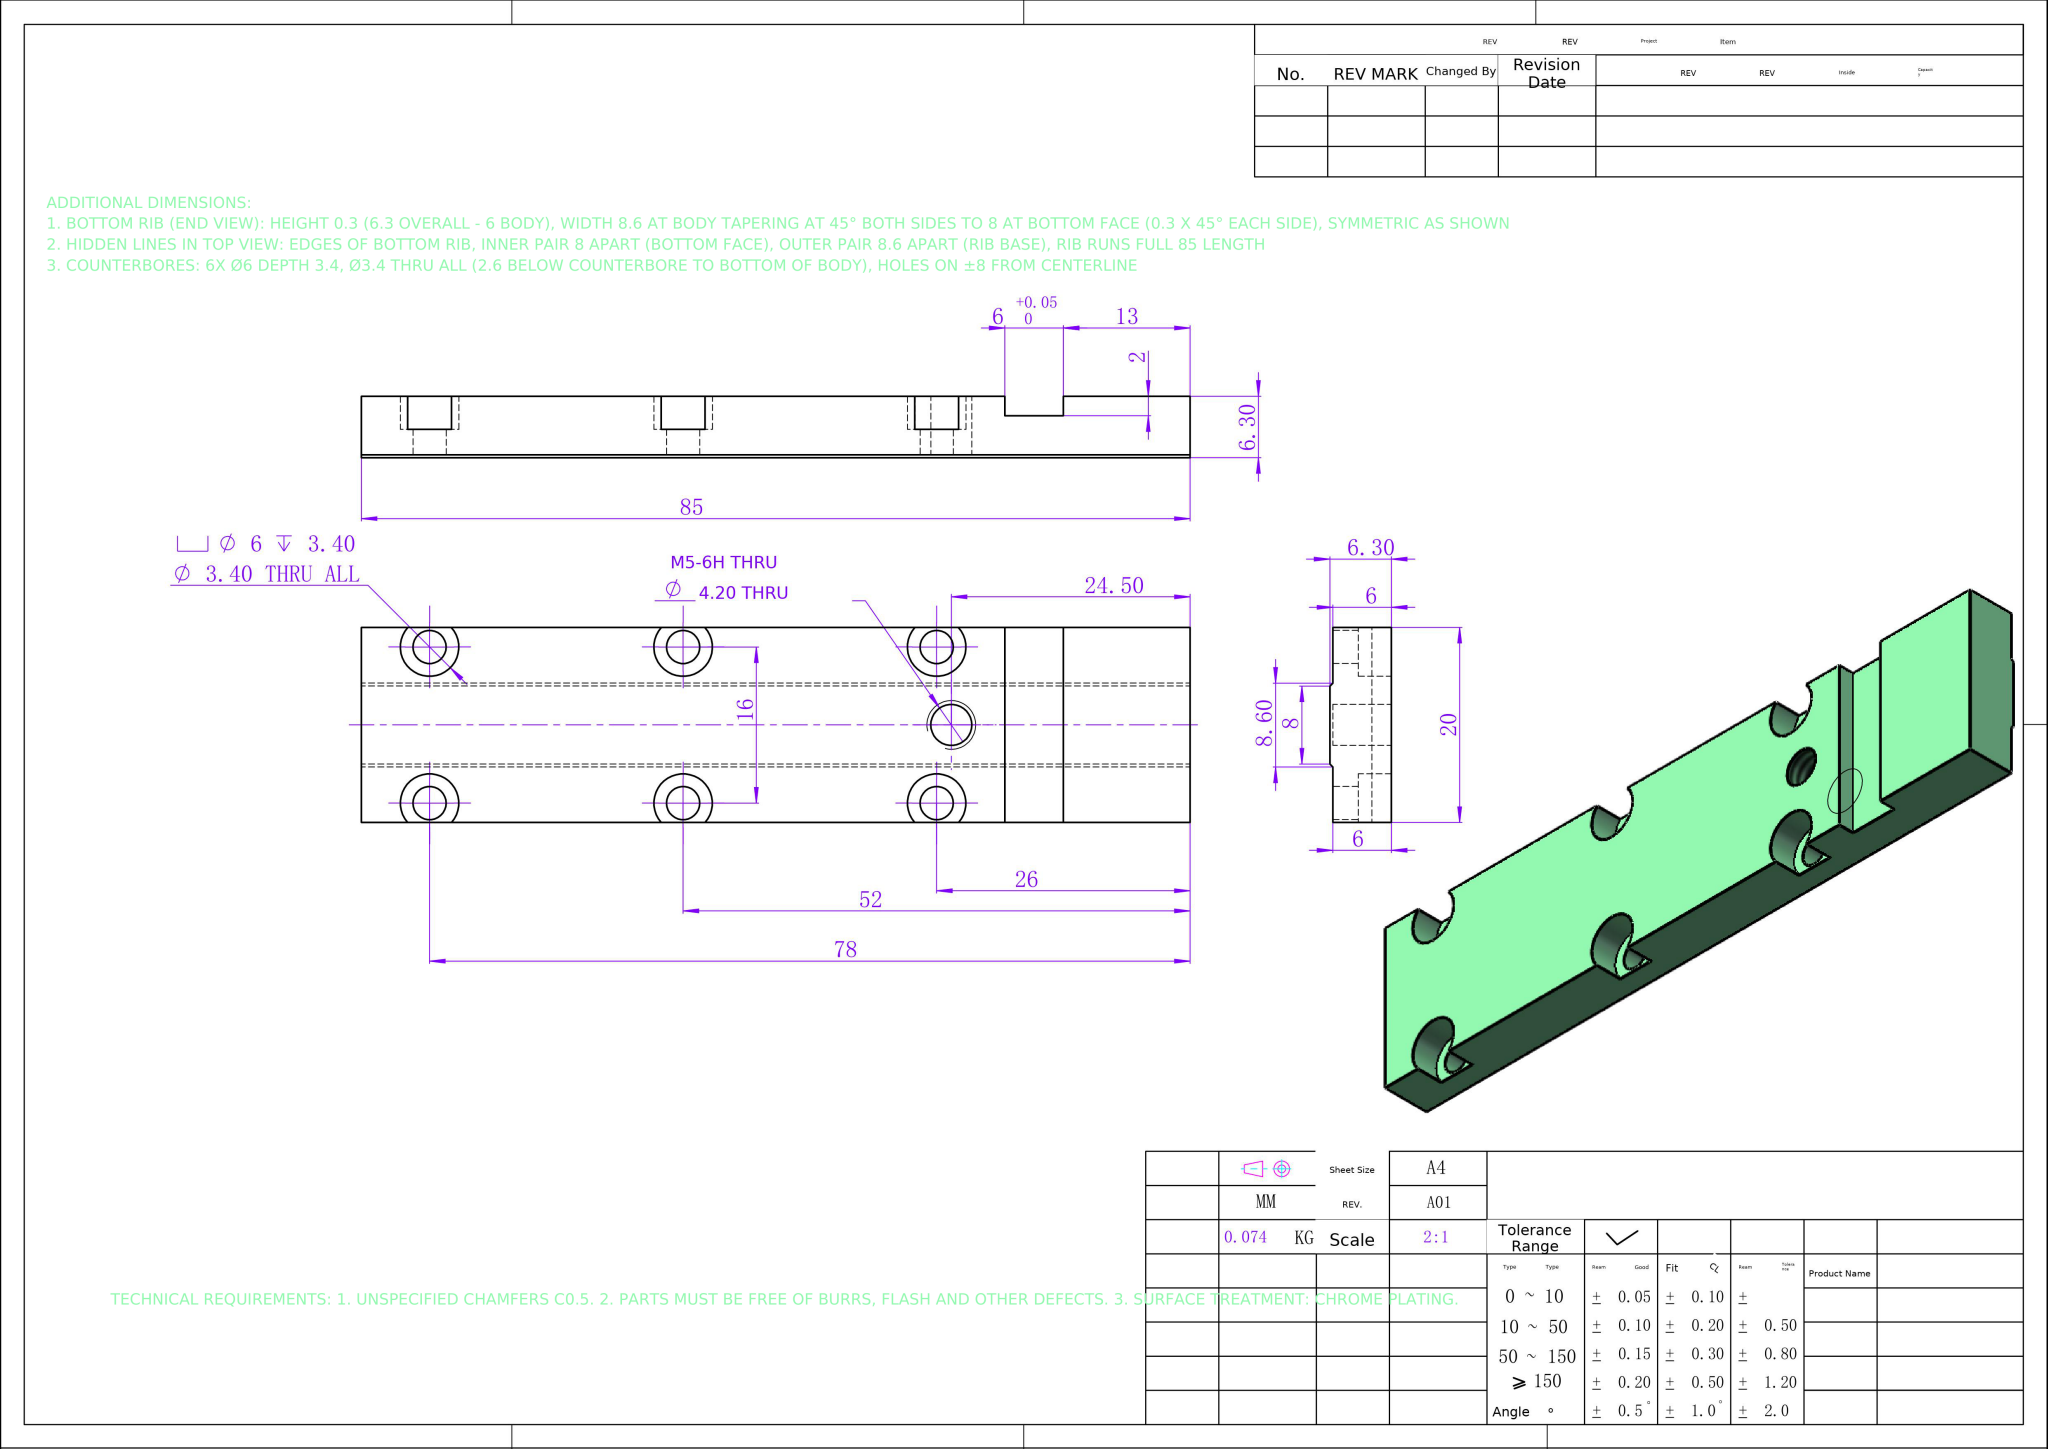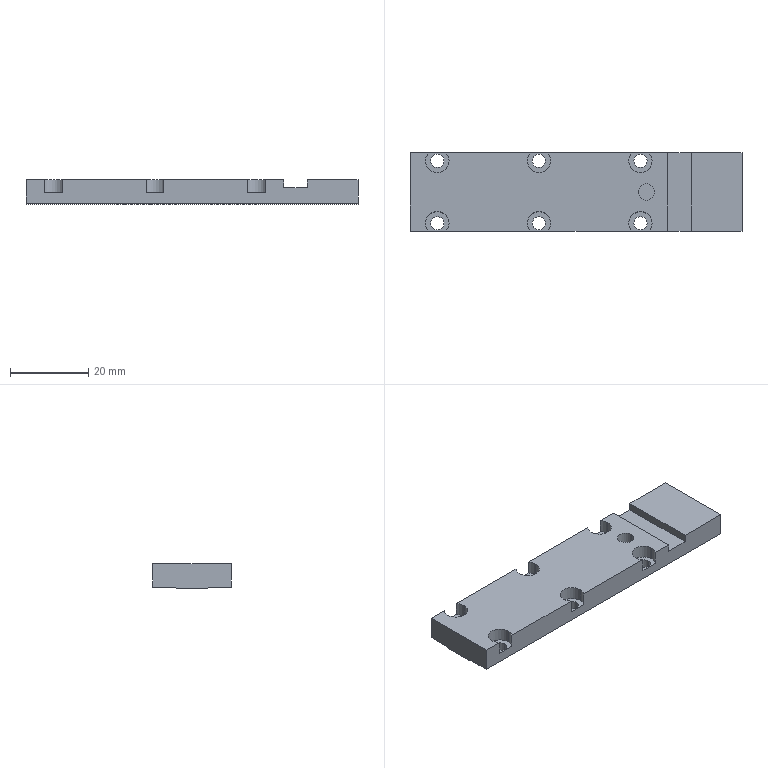Part | NX | mm | 1 solid | 53 faces | box 85 x 20 x 6.3 mm | volume 9433 mm3 | cylinder 32 | plane 21 | commonest cylinder face diameters 6 x18 3.4 x12 4.2 x2